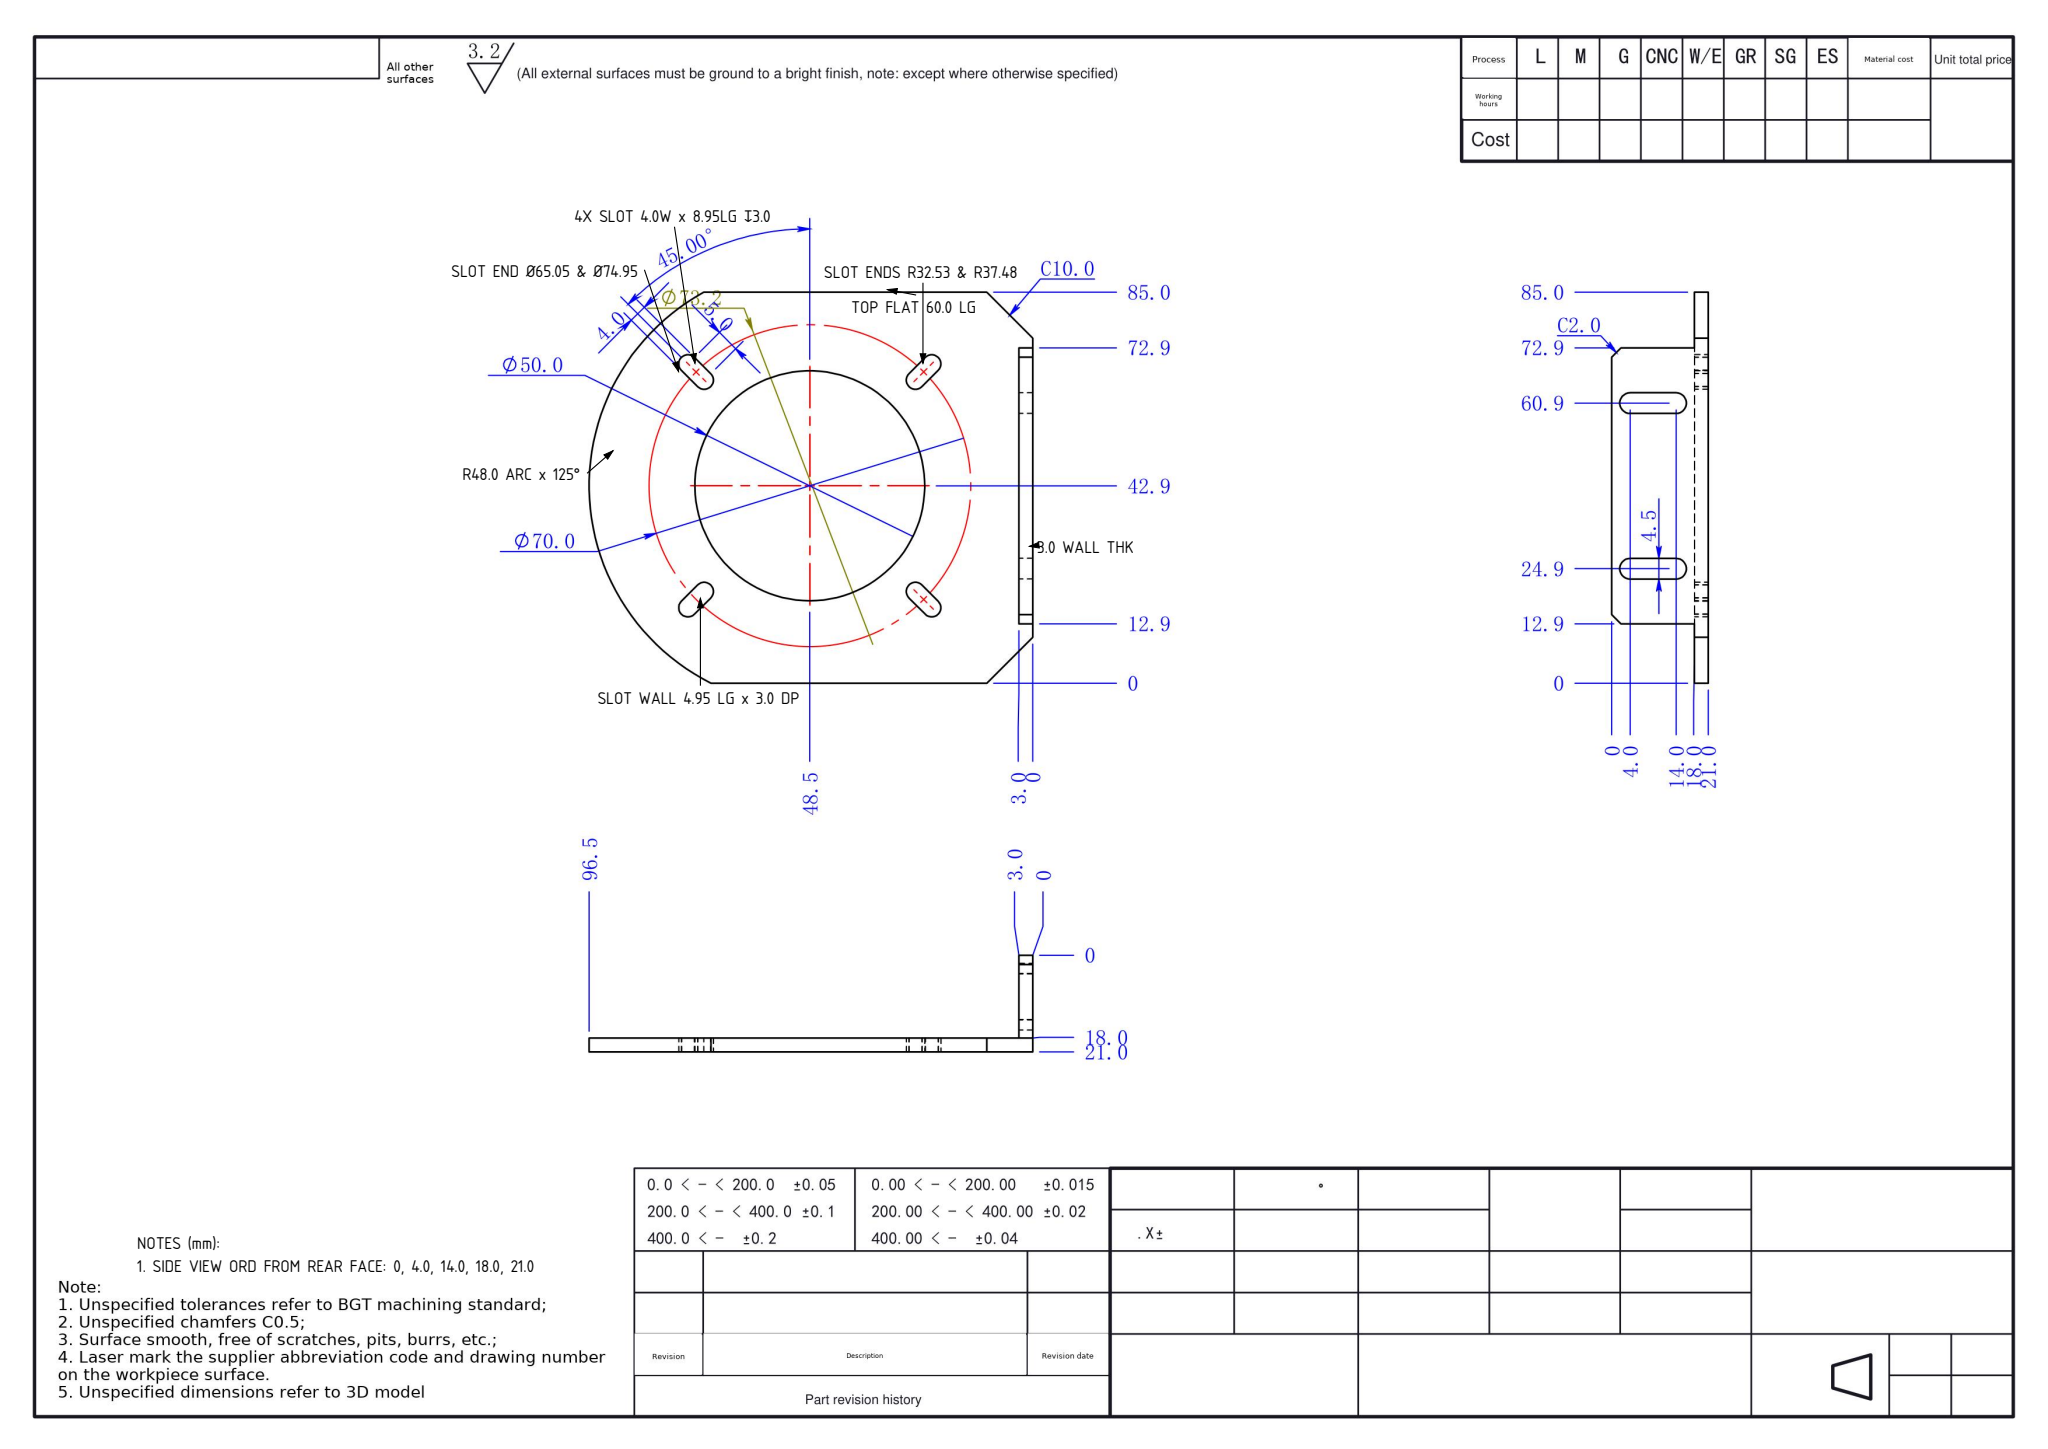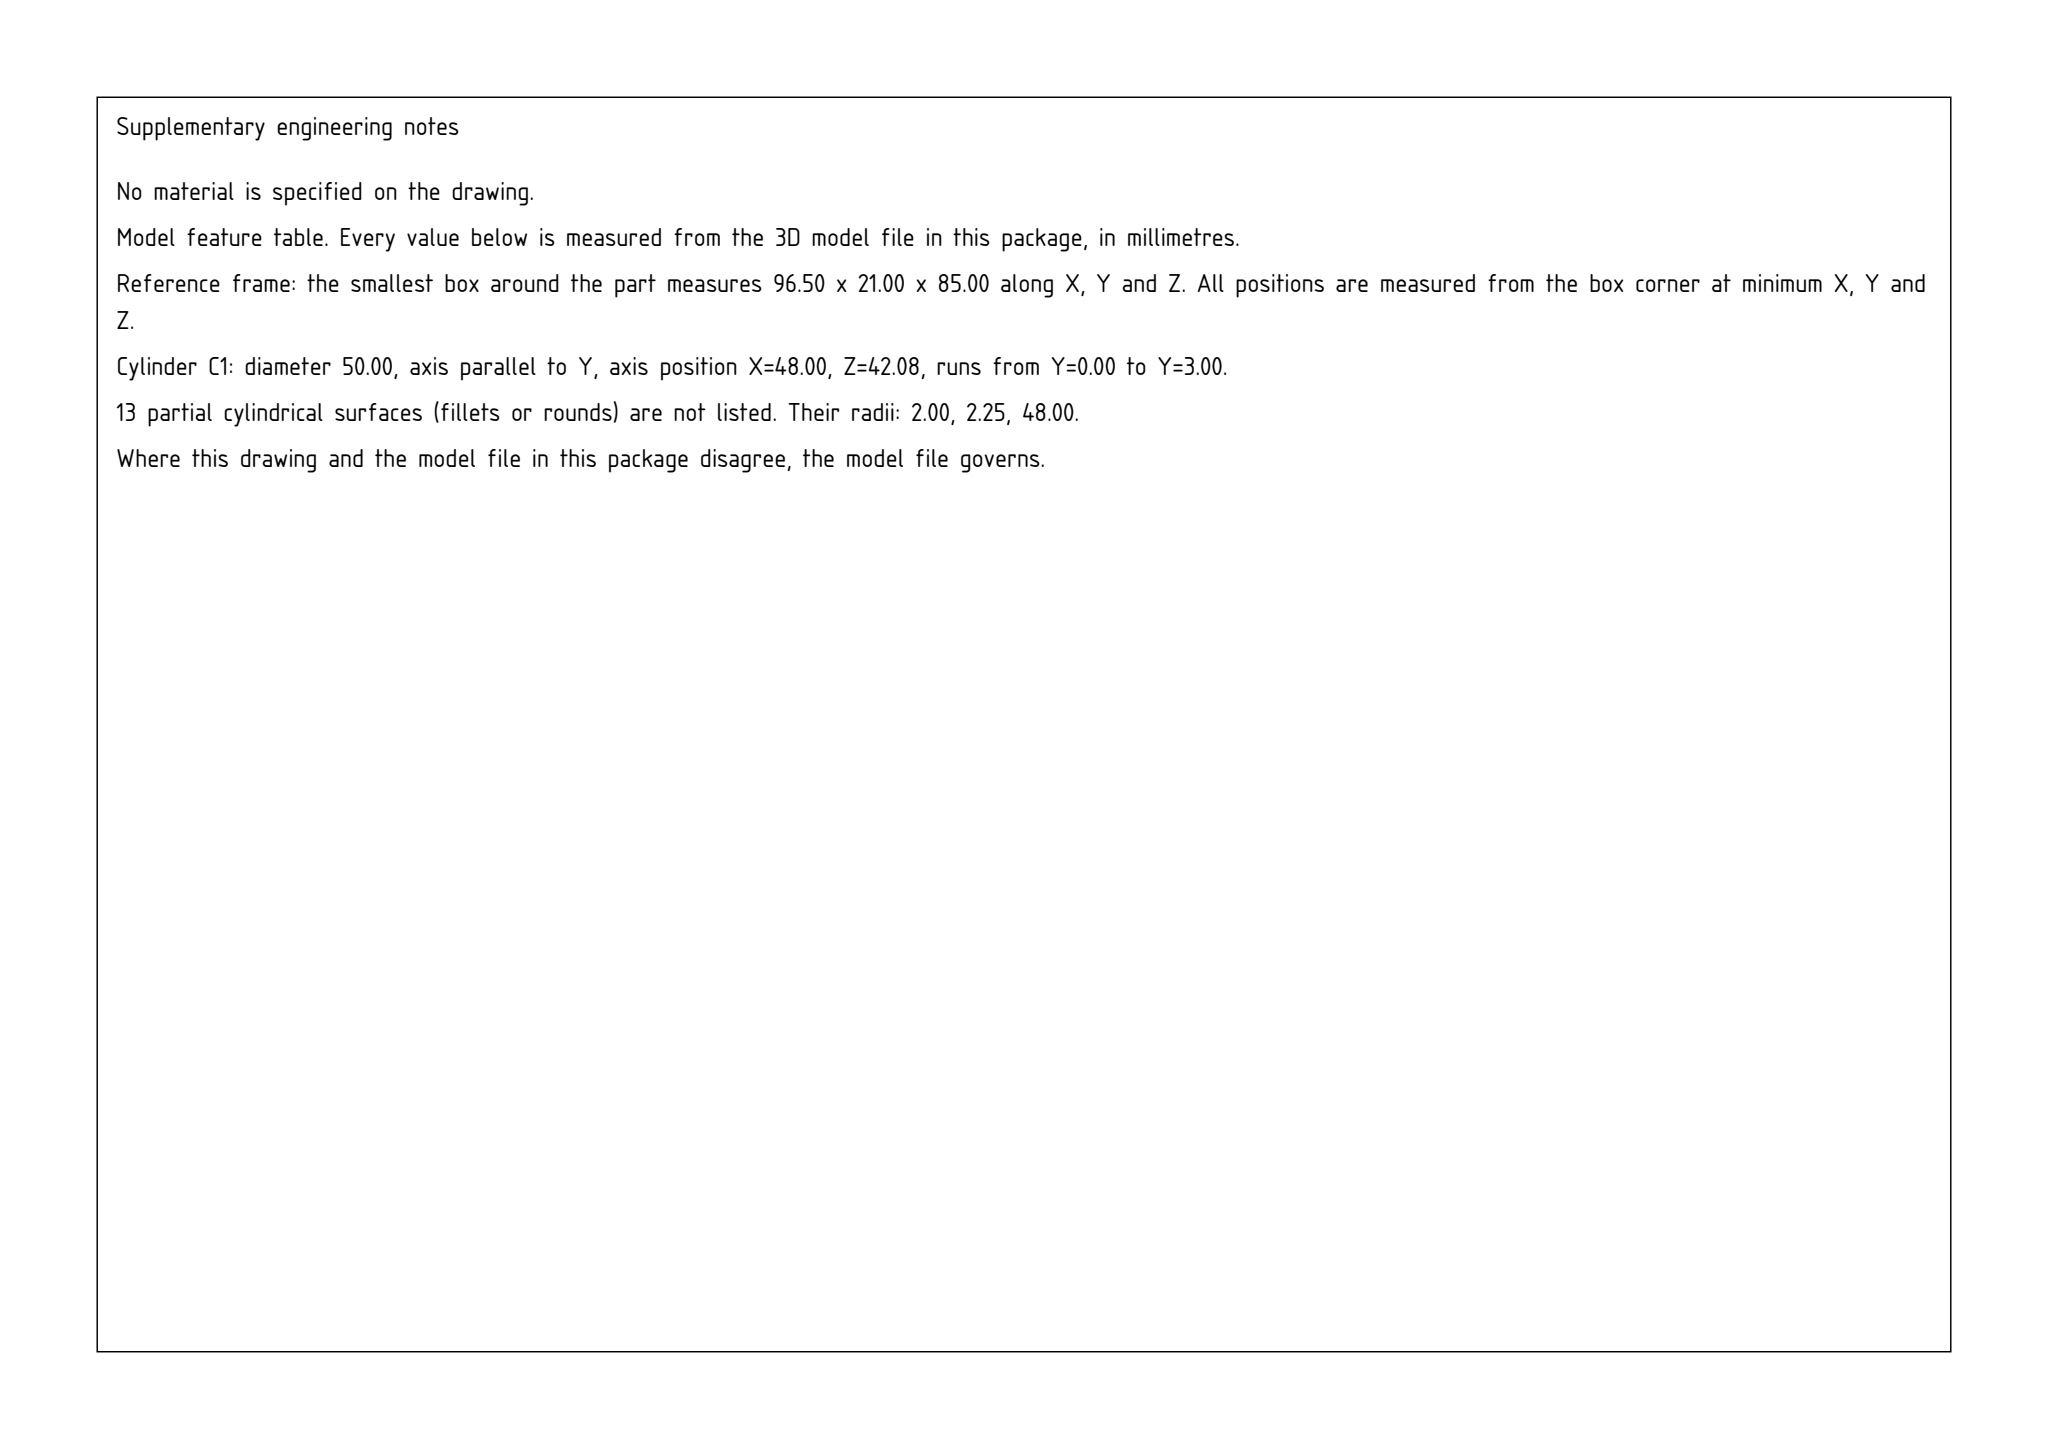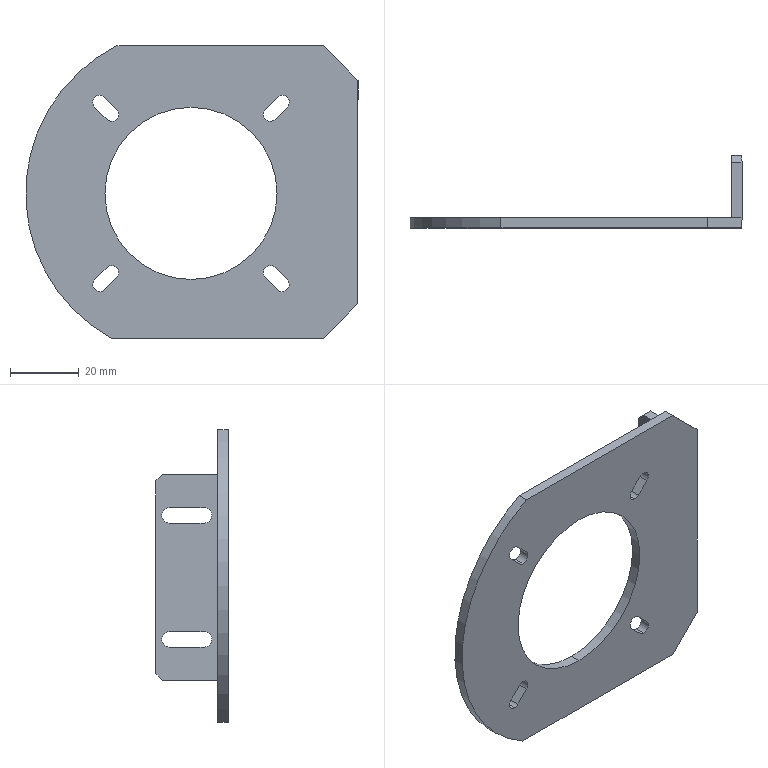Part | SolidWorks | mm | 1 solid | 44 faces | box 96.5 x 21 x 85 mm | volume 19008 mm3 | plane 25 | cylinder 19 | commonest cylinder face diameters 4 x12 4.5 x4 50 x2 96 x1
Drawing notes:
OUTER PROFILE ARC R48.0 (Ø96.0) x 125°, CTR ON Ø50.0 BORE CL | from the solid: convex arc dia 96.0 axis y at (x48.0,z42.1), arc_deg 125; Ø50.0 bore same axis
4X RAD SLOT 4.0 W x 8.95 LG, ENDS Ø61.05 & Ø78.95, THRU 3.0 | from the solid: slot end arcs Ø4.0 at r32.53 & r37.48 from (48.0,42.1), y 0-3.0; 8 side planes 45° 3.5x3.5
TOP FLAT 60.0 LG, BOT FLAT 61.6 LG, TAN TO R48.0 ARC | from the solid: plane z=85.0 x 26.5-86.5; plane z=0 x 24.9-86.5; arc R48 ctr x48.0 z42.1
UPPER-LEFT Ø: BC Ø70.0, SLOT END CTRS Ø65.05 & Ø74.95 | from the solid: slot end arc centers at r32.53 and r37.48 (mid r35.0 = Ø70.0 BC)
FRONT VIEW RH ORD = 0 & 3.0 (RH WALL 3.0 THK), NOT 3.8 | from the solid: planes x=93.5 and x=96.5, 3.0 apart
SIDE VIEW ORD FROM REAR FACE: 0, 4.0, 14.0, 18.0, 21.0 | from the solid: y faces at 21.0,17.0,7.0,3.0,0.0 -> 0,4.0,14.0,18.0,21.0 from y=21.0
4X SLOT 4.0 WIDE x 8.95 LONG THRU 3.0 PLATE; SLOT END ARC CTRS AT R32.53 AND R37.48 FROM Ø50.0 BORE CL, EACH SLOT AXIS RADIAL AT 45° TO PART AXES | from the solid: cylinders: 8X concave arc dia 4.0, axis y, from 0.0 to 3.0 at (21.5,15.6),(25.0,19.1),(71.0,19.1),(74.5,15.6),(21.5,68.6),(25.0,65.1),(71.0,65.1),(74.5,68.6); bore 50.0 axis y at (48.0,42.1)
SLOT SIDE WALLS ARE FLAT FACES 4.95 LONG x 3.0 DEEP, AT 45° TO X AND Z AXES (8 PLACES) | from the solid: inclined_planes 45/90/45, size [3.5,3.0,3.5] at bbox_from (20.1,0,17.0),(22.9,0,14.2),(69.6,0,14.2),(72.4,0,17.0),(20.1,0,63.7),(22.9,0,66.5),(69.6,0,66.5),(72.4,0,63.7)
build123d program:
from build123d import *

# Parameters (mm, degrees)
SKETCH3_R           = 25
BOSS_EXTRUDE2_DEPTH = 3
SKETCH4_W           = 3
SKETCH4_H           = 85
BOSS_EXTRUDE3_DEPTH = 18
SKETCH5_W           = 12.891
SKETCH5_H           = 18
SKETCH5_W_2         = 12.109
CUT_EXTRUDE1_DEPTH  = 129.441
CUT_EXTRUDE2_DEPTH  = 50
SKETCH7_R           = 1.75
CUT_EXTRUDE3_DEPTH  = 90
CHAMFER1_SIZE       = 10
CHAMFER2_SIZE       = 2
CUT_EXTRUDE5_DEPTH  = 112.596
CIRPATTERN1_COUNT   = 4


with BuildPart() as part:
    # Sketch3 → Boss-Extrude2 (new body)
    with BuildSketch(Plane(origin=(0, 0, 0), x_dir=(1, 0, 0), z_dir=(0, 1, 0))):
        with BuildLine():
            Line((-1.451, 0.5207), (68.549, 0.5207))
            Line((68.549, 0.5207), (68.549, 85.521))
            Line((68.549, 85.521), (-3.036, 85.521))
            ThreePointArc((-3.036, 85.521), (-27.943, 42.542), (-1.451, 0.5207))
        make_face()
        with Locations(Location((20.049, 43.436, 0), (0, 0, 270))):
            Circle(SKETCH3_R, mode=Mode.SUBTRACT)
    extrude(amount=BOSS_EXTRUDE2_DEPTH)

    # Sketch4 → Boss-Extrude3 (add)
    with BuildSketch(Plane(origin=(0, 3, 0), x_dir=(1, 0, 0), z_dir=(0, 1, 0))):
        with Locations((67.049, 43.021)):
            Rectangle(SKETCH4_W, SKETCH4_H)
    extrude(amount=BOSS_EXTRUDE3_DEPTH)

    # Sketch5 → Cut-Extrude1 (cut, through all)
    with BuildSketch(Plane.ZY.offset(-65.549)):
        with Locations((-6.966, 12)):
            Rectangle(SKETCH5_W, SKETCH5_H)
        with Locations((-79.466, 12)):
            Rectangle(SKETCH5_W_2, SKETCH5_H)
    extrude(amount=-CUT_EXTRUDE1_DEPTH, mode=Mode.SUBTRACT)

    # Sketch6 → Cut-Extrude2 (cut)
    with BuildSketch(Plane(origin=(68.549, 0, 0), x_dir=(0, 0, -1), z_dir=(1, 0, 0))):
        with BuildLine():
            Line((27.662, 17), (27.662, 7))
            ThreePointArc((27.662, 7), (25.412, 4.75), (23.162, 7))
            Line((23.162, 7), (23.162, 17))
            ThreePointArc((23.162, 17), (25.412, 19.25), (27.662, 17))
        make_face()
        with BuildLine():
            Line((59.162, 17), (59.162, 7))
            ThreePointArc((59.162, 7), (61.412, 4.75), (63.662, 7))
            Line((63.662, 7), (63.662, 17))
            ThreePointArc((63.662, 17), (61.412, 19.25), (59.162, 17))
        make_face()
    extrude(amount=-CUT_EXTRUDE2_DEPTH, mode=Mode.SUBTRACT)

    # Sketch7 → Cut-Extrude3 (cut)
    with BuildSketch(Plane(origin=(0, 3, 0), x_dir=(1, 0, 0), z_dir=(0, 1, 0))):
        with Locations(Location((-4.7, 68.185, 0), (0, 0, 270))):
            Circle(SKETCH7_R)
        with Locations(Location((44.798, 68.185, 0), (0, 0, 270))):
            Circle(SKETCH7_R)
        with Locations(Location((44.798, 18.688, 0), (0, 0, 270))):
            Circle(SKETCH7_R)
        with Locations(Location((-4.7, 18.688, 0), (0, 0, 270))):
            Circle(SKETCH7_R)
    extrude(amount=-CUT_EXTRUDE3_DEPTH, mode=Mode.SUBTRACT)

    # Chamfer1
    chamfer1_edges = [part.edges().sort_by_distance(p)[0] for p in [
        (68.549, 1.5, -85.521),
        (68.549, 1.5, -0.5207),
    ]]
    chamfer(chamfer1_edges, length=CHAMFER1_SIZE)

    # Chamfer2
    chamfer2_edges = [part.edges().sort_by_distance(p)[0] for p in [
        (67.049, 21, -13.412),
        (67.049, 21, -73.412),
    ]]
    chamfer(chamfer2_edges, length=CHAMFER2_SIZE)

    # Sketch9 → Cut-Extrude5 (cut, through all)
    with BuildSketch(Plane.XZ):
        with BuildLine():
            Line((-4.346, -21.87), (-7.882, -18.334))
            ThreePointArc((-7.882, -18.334), (-7.882, -15.506), (-5.053, -15.506))
            Line((-5.053, -15.506), (-1.518, -19.041))
            ThreePointArc((-1.518, -19.041), (-1.518, -21.87), (-4.346, -21.87))
        make_face()
    cut_extrude5 = extrude(amount=-CUT_EXTRUDE5_DEPTH, mode=Mode.SUBTRACT)

    # CirPattern1: Cut-Extrude5 ×4 about axis
    cirpattern1_axis = Axis((20.049, 0, -43.436), (0, 1, 0))
    for i in range(1, CIRPATTERN1_COUNT):
        add(cut_extrude5.rotate(cirpattern1_axis, i * 360 / CIRPATTERN1_COUNT), mode=Mode.SUBTRACT)


solid = part.part